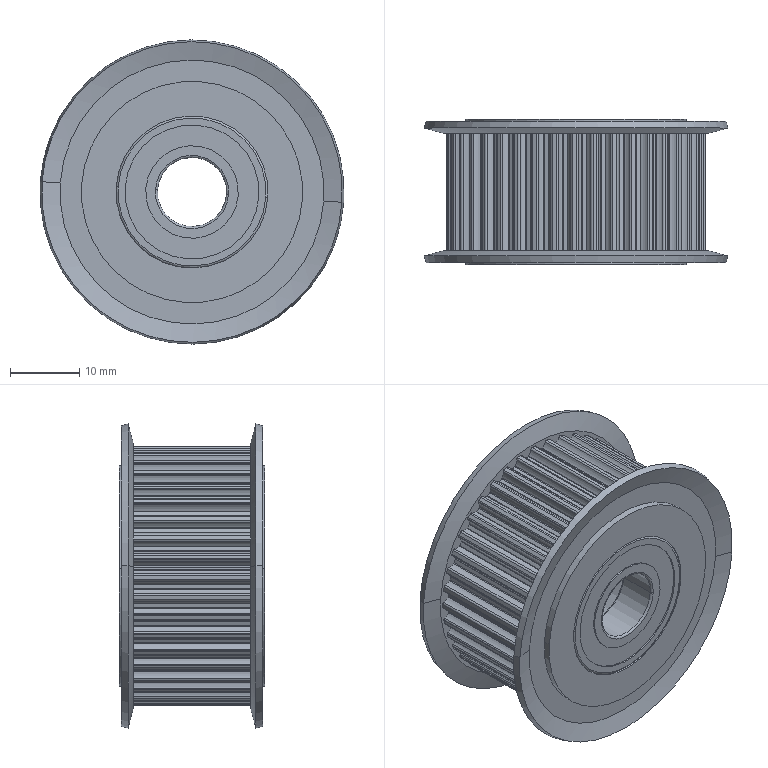Component | SolidWorks | EVD21-40-S3M150.stp-1 | 1 solid | 439 faces | volume 18335 mm3 | cylinder 391 | plane 20 | torus 16 | cone 12 | commonest cylinder face diameters 0.56 x98 0.3 x90 3.95 x88 35.22 x41 37.44 x40 13.4 x8 19.4 x8 22 x8 | material 6061 Alloy